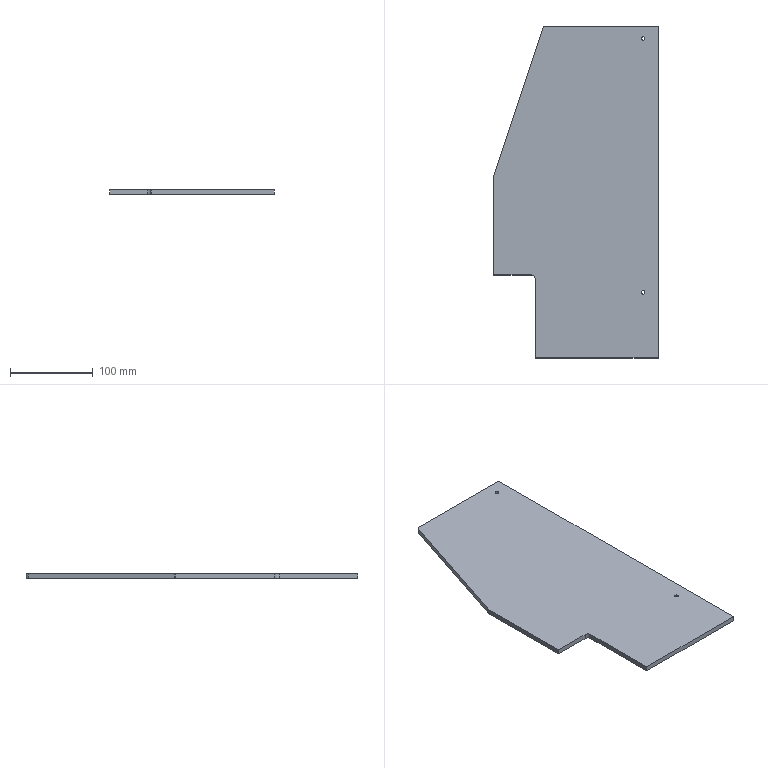Component | SolidWorks | THK-B1005LeftFrontBaffle-1 | 1 solid | 16 faces | box 198 x 400 x 6 mm | volume 412657 mm3 | plane 9 | cylinder 7 | commonest cylinder face diameters 4.2 x4 8 x2 10 x1 | material Q235A
build123d program:
from build123d import *

# Parameters (mm, degrees)
BOSS_EXTRUDE1_DEPTH = 3
M5_TAPPED_HOLE1_D   = 4.2
FILLET1_R           = 4


with BuildPart() as part:
    # Sketch1 → Boss-Extrude1 (new, symmetric)
    with BuildSketch(Plane.XY):
        with BuildLine():
            Line((-39, 200), (99, 200))
            Line((99, 200), (99, -200))
            Line((99, -200), (-49, -200))
            Line((-49, -200), (-49, -105))
            ThreePointArc((-49, -105), (-50.464, -101.464), (-54, -100))
            Line((-54, -100), (-99, -100))
            Line((-99, -100), (-99, 20))
            Line((-99, 20), (-39, 200))
        make_face()
    extrude(amount=BOSS_EXTRUDE1_DEPTH, both=True)

    # M5 Tapped Hole1 (through all)
    with Locations(Plane.XY.offset(3)):
        with Locations((81, 185), (81, -121)):
            Hole(M5_TAPPED_HOLE1_D / 2)

    # Fillet1
    fillet1_edges = [part.edges().sort_by_distance(p)[0] for p in [
        (-99, 20, 0),
        (-39, 200, 0),
    ]]
    fillet(fillet1_edges, radius=FILLET1_R)


solid = part.part

# Placed as in the assembly
solid = solid.moved(Location((-221, 0, -258), (0, 0, 0)))
STEP:
#1=COLOUR_RGB('',0.7922,0.8196,0.9333);
#2=FILL_AREA_STYLE_COLOUR('',#1);
#3=FILL_AREA_STYLE('',(#2));
#4=SURFACE_STYLE_FILL_AREA(#3);
#5=SURFACE_SIDE_STYLE('',(#4));
#6=SURFACE_STYLE_USAGE(.BOTH.,#5);
#7=PRESENTATION_STYLE_ASSIGNMENT((#6));
#8=CARTESIAN_POINT('',(-5.594,7.283,-10.276));
#9=VERTEX_POINT('',#8);
#10=CARTESIAN_POINT('',(-5.429,7.283,-10.276));
#11=VERTEX_POINT('',#10);
#12=CARTESIAN_POINT('',(-5.512,7.283,-10.276));
#13=DIRECTION('',(0.,0.,1.));
#14=DIRECTION('',(1.,0.,0.));
#15=AXIS2_PLACEMENT_3D('',#12,#13,#14);
#16=CIRCLE('',#15,0.08268);
#17=EDGE_CURVE('',#9,#11,#16,.T.);
#18=ORIENTED_EDGE('',*,*,#17,.F.);
#19=CARTESIAN_POINT('',(-5.594,7.283,-10.039));
#20=VERTEX_POINT('',#19);
#21=CARTESIAN_POINT('',(-5.594,7.283,-10.039));
#22=DIRECTION('',(0.,0.,1.));
#23=VECTOR('',#22,39.37);
#24=LINE('',#21,#23);
#25=EDGE_CURVE('',#9,#20,#24,.T.);
#26=ORIENTED_EDGE('',*,*,#25,.T.);
#27=CARTESIAN_POINT('',(-5.429,7.283,-10.039));
#28=VERTEX_POINT('',#27);
#29=CARTESIAN_POINT('',(-5.512,7.283,-10.039));
#30=DIRECTION('',(0.,0.,1.));
#31=DIRECTION('',(1.,0.,0.));
#32=AXIS2_PLACEMENT_3D('',#29,#30,#31);
#33=CIRCLE('',#32,0.08268);
#34=EDGE_CURVE('',#20,#28,#33,.T.);
#35=ORIENTED_EDGE('',*,*,#34,.T.);
#36=CARTESIAN_POINT('',(-5.429,7.283,-10.039));
#37=DIRECTION('',(0.,0.,1.));
#38=VECTOR('',#37,39.37);
#39=LINE('',#36,#38);
#40=EDGE_CURVE('',#11,#28,#39,.T.);
#41=ORIENTED_EDGE('',*,*,#40,.F.);
#42=EDGE_LOOP('',(#18,#26,#35,#41));
#43=FACE_OUTER_BOUND('',#42,.T.);
#44=CARTESIAN_POINT('',(-5.512,7.283,-10.039));
#45=DIRECTION('',(0.,0.,1.));
#46=DIRECTION('',(1.,0.,0.));
#47=AXIS2_PLACEMENT_3D('',#44,#45,#46);
#48=CYLINDRICAL_SURFACE('',#47,0.08268);
#49=ADVANCED_FACE('',(#43),#48,.F.);
#50=CARTESIAN_POINT('',(-5.594,-4.764,-10.276));
#51=VERTEX_POINT('',#50);
#52=CARTESIAN_POINT('',(-5.429,-4.764,-10.276));
#53=VERTEX_POINT('',#52);
#54=CARTESIAN_POINT('',(-5.512,-4.764,-10.276));
#55=DIRECTION('',(0.,0.,1.));
#56=DIRECTION('',(1.,0.,0.));
#57=AXIS2_PLACEMENT_3D('',#54,#55,#56);
#58=CIRCLE('',#57,0.08268);
#59=EDGE_CURVE('',#51,#53,#58,.T.);
#60=ORIENTED_EDGE('',*,*,#59,.F.);
#61=CARTESIAN_POINT('',(-5.594,-4.764,-10.039));
#62=VERTEX_POINT('',#61);
#63=CARTESIAN_POINT('',(-5.594,-4.764,-10.039));
#64=DIRECTION('',(0.,0.,1.));
#65=VECTOR('',#64,39.37);
#66=LINE('',#63,#65);
#67=EDGE_CURVE('',#51,#62,#66,.T.);
#68=ORIENTED_EDGE('',*,*,#67,.T.);
#69=CARTESIAN_POINT('',(-5.429,-4.764,-10.039));
#70=VERTEX_POINT('',#69);
#71=CARTESIAN_POINT('',(-5.512,-4.764,-10.039));
#72=DIRECTION('',(0.,0.,1.));
#73=DIRECTION('',(1.,0.,0.));
#74=AXIS2_PLACEMENT_3D('',#71,#72,#73);
#75=CIRCLE('',#74,0.08268);
#76=EDGE_CURVE('',#62,#70,#75,.T.);
#77=ORIENTED_EDGE('',*,*,#76,.T.);
#78=CARTESIAN_POINT('',(-5.429,-4.764,-10.039));
#79=DIRECTION('',(0.,0.,1.));
#80=VECTOR('',#79,39.37);
#81=LINE('',#78,#80);
#82=EDGE_CURVE('',#53,#70,#81,.T.);
#83=ORIENTED_EDGE('',*,*,#82,.F.);
#84=EDGE_LOOP('',(#60,#68,#77,#83));
#85=FACE_OUTER_BOUND('',#84,.T.);
#86=CARTESIAN_POINT('',(-5.512,-4.764,-10.039));
#87=DIRECTION('',(0.,0.,1.));
#88=DIRECTION('',(1.,0.,0.));
#89=AXIS2_PLACEMENT_3D('',#86,#87,#88);
#90=CYLINDRICAL_SURFACE('',#89,0.08268);
#91=ADVANCED_FACE('',(#85),#90,.F.);
#92=CARTESIAN_POINT('',(-12.598,0.7618,-10.039));
#93=VERTEX_POINT('',#92);
#94=CARTESIAN_POINT('',(-12.598,-3.937,-10.039));
#95=VERTEX_POINT('',#94);
#96=CARTESIAN_POINT('',(-12.598,0.7874,-10.039));
#97=DIRECTION('',(0.,-1.,0.));
#98=VECTOR('',#97,39.37);
#99=LINE('',#96,#98);
#100=EDGE_CURVE('',#93,#95,#99,.T.);
#101=ORIENTED_EDGE('',*,*,#100,.F.);
#102=CARTESIAN_POINT('',(-12.598,0.7618,-10.276));
#103=VERTEX_POINT('',#102);
#104=CARTESIAN_POINT('',(-12.598,0.7618,-10.039));
#105=DIRECTION('',(0.,0.,-1.));
#106=VECTOR('',#105,39.37);
#107=LINE('',#104,#106);
#108=EDGE_CURVE('',#93,#103,#107,.T.);
#109=ORIENTED_EDGE('',*,*,#108,.T.);
#110=CARTESIAN_POINT('',(-12.598,-3.937,-10.276));
#111=VERTEX_POINT('',#110);
#112=CARTESIAN_POINT('',(-12.598,0.7874,-10.276));
#113=DIRECTION('',(0.,-1.,0.));
#114=VECTOR('',#113,39.37);
#115=LINE('',#112,#114);
#116=EDGE_CURVE('',#103,#111,#115,.T.);
#117=ORIENTED_EDGE('',*,*,#116,.T.);
#118=CARTESIAN_POINT('',(-12.598,-3.937,-10.039));
#119=DIRECTION('',(0.,0.,-1.));
#120=VECTOR('',#119,39.37);
#121=LINE('',#118,#120);
#122=EDGE_CURVE('',#95,#111,#121,.T.);
#123=ORIENTED_EDGE('',*,*,#122,.F.);
#124=EDGE_LOOP('',(#101,#109,#117,#123));
#125=FACE_OUTER_BOUND('',#124,.T.);
#126=CARTESIAN_POINT('',(-12.598,0.7874,-10.039));
#127=DIRECTION('',(1.,0.,0.));
#128=DIRECTION('',(0.,0.,-1.));
#129=AXIS2_PLACEMENT_3D('',#126,#127,#128);
#130=PLANE('',#129);
#131=ADVANCED_FACE('',(#125),#130,.F.);
#132=CARTESIAN_POINT('',(-10.827,-3.937,-10.276));
#133=VERTEX_POINT('',#132);
#134=CARTESIAN_POINT('',(-10.827,-3.937,-10.276));
#135=DIRECTION('',(1.,0.,0.));
#136=VECTOR('',#135,39.37);
#137=LINE('',#134,#136);
#138=EDGE_CURVE('',#111,#133,#137,.T.);
#139=ORIENTED_EDGE('',*,*,#138,.T.);
#140=CARTESIAN_POINT('',(-10.827,-3.937,-10.039));
#141=VERTEX_POINT('',#140);
#142=CARTESIAN_POINT('',(-10.827,-3.937,-10.039));
#143=DIRECTION('',(0.,0.,-1.));
#144=VECTOR('',#143,39.37);
#145=LINE('',#142,#144);
#146=EDGE_CURVE('',#141,#133,#145,.T.);
#147=ORIENTED_EDGE('',*,*,#146,.F.);
#148=CARTESIAN_POINT('',(-10.827,-3.937,-10.039));
#149=DIRECTION('',(1.,0.,0.));
#150=VECTOR('',#149,39.37);
#151=LINE('',#148,#150);
#152=EDGE_CURVE('',#95,#141,#151,.T.);
#153=ORIENTED_EDGE('',*,*,#152,.F.);
#154=ORIENTED_EDGE('',*,*,#122,.T.);
#155=EDGE_LOOP('',(#139,#147,#153,#154));
#156=FACE_OUTER_BOUND('',#155,.T.);
#157=CARTESIAN_POINT('',(-10.827,-3.937,-10.039));
#158=DIRECTION('',(-0.,1.,0.));
#159=DIRECTION('',(-1.,-0.,0.));
#160=AXIS2_PLACEMENT_3D('',#157,#158,#159);
#161=PLANE('',#160);
#162=ADVANCED_FACE('',(#156),#161,.F.);
#163=CARTESIAN_POINT('',(-10.63,-4.134,-10.276));
#164=VERTEX_POINT('',#163);
#165=CARTESIAN_POINT('',(-10.827,-4.134,-10.276));
#166=DIRECTION('',(0.,0.,-1.));
#167=DIRECTION('',(1.,0.,0.));
#168=AXIS2_PLACEMENT_3D('',#165,#166,#167);
#169=CIRCLE('',#168,0.1969);
#170=EDGE_CURVE('',#133,#164,#169,.T.);
#171=ORIENTED_EDGE('',*,*,#170,.T.);
#172=CARTESIAN_POINT('',(-10.63,-4.134,-10.039));
#173=VERTEX_POINT('',#172);
#174=CARTESIAN_POINT('',(-10.63,-4.134,-10.039));
#175=DIRECTION('',(0.,0.,-1.));
#176=VECTOR('',#175,39.37);
#177=LINE('',#174,#176);
#178=EDGE_CURVE('',#173,#164,#177,.T.);
#179=ORIENTED_EDGE('',*,*,#178,.F.);
#180=CARTESIAN_POINT('',(-10.827,-4.134,-10.039));
#181=DIRECTION('',(0.,0.,-1.));
#182=DIRECTION('',(1.,0.,0.));
#183=AXIS2_PLACEMENT_3D('',#180,#181,#182);
#184=CIRCLE('',#183,0.1969);
#185=EDGE_CURVE('',#141,#173,#184,.T.);
#186=ORIENTED_EDGE('',*,*,#185,.F.);
#187=ORIENTED_EDGE('',*,*,#146,.T.);
#188=EDGE_LOOP('',(#171,#179,#186,#187));
#189=FACE_OUTER_BOUND('',#188,.T.);
#190=CARTESIAN_POINT('',(-10.827,-4.134,-10.039));
#191=DIRECTION('',(0.,0.,-1.));
#192=DIRECTION('',(-1.,0.,0.));
#193=AXIS2_PLACEMENT_3D('',#190,#191,#192);
#194=CYLINDRICAL_SURFACE('',#193,0.1969);
#195=ADVANCED_FACE('',(#189),#194,.F.);
#196=CARTESIAN_POINT('',(-10.63,-7.874,-10.276));
#197=VERTEX_POINT('',#196);
#198=CARTESIAN_POINT('',(-10.63,-7.874,-10.276));
#199=DIRECTION('',(0.,-1.,0.));
#200=VECTOR('',#199,39.37);
#201=LINE('',#198,#200);
#202=EDGE_CURVE('',#164,#197,#201,.T.);
#203=ORIENTED_EDGE('',*,*,#202,.T.);
#204=CARTESIAN_POINT('',(-10.63,-7.874,-10.039));
#205=VERTEX_POINT('',#204);
#206=CARTESIAN_POINT('',(-10.63,-7.874,-10.039));
#207=DIRECTION('',(0.,0.,-1.));
#208=VECTOR('',#207,39.37);
#209=LINE('',#206,#208);
#210=EDGE_CURVE('',#205,#197,#209,.T.);
#211=ORIENTED_EDGE('',*,*,#210,.F.);
#212=CARTESIAN_POINT('',(-10.63,-7.874,-10.039));
#213=DIRECTION('',(0.,-1.,0.));
#214=VECTOR('',#213,39.37);
#215=LINE('',#212,#214);
#216=EDGE_CURVE('',#173,#205,#215,.T.);
#217=ORIENTED_EDGE('',*,*,#216,.F.);
#218=ORIENTED_EDGE('',*,*,#178,.T.);
#219=EDGE_LOOP('',(#203,#211,#217,#218));
#220=FACE_OUTER_BOUND('',#219,.T.);
#221=CARTESIAN_POINT('',(-10.63,-7.874,-10.039));
#222=DIRECTION('',(1.,0.,0.));
#223=DIRECTION('',(0.,0.,-1.));
#224=AXIS2_PLACEMENT_3D('',#221,#222,#223);
#225=PLANE('',#224);
#226=ADVANCED_FACE('',(#220),#225,.F.);
#227=CARTESIAN_POINT('',(-4.803,-7.874,-10.276));
#228=VERTEX_POINT('',#227);
#229=CARTESIAN_POINT('',(-10.63,-7.874,-10.276));
#230=DIRECTION('',(1.,0.,0.));
#231=VECTOR('',#230,39.37);
#232=LINE('',#229,#231);
#233=EDGE_CURVE('',#197,#228,#232,.T.);
#234=ORIENTED_EDGE('',*,*,#233,.T.);
#235=CARTESIAN_POINT('',(-4.803,-7.874,-10.039));
#236=VERTEX_POINT('',#235);
#237=CARTESIAN_POINT('',(-4.803,-7.874,-10.039));
#238=DIRECTION('',(0.,0.,-1.));
#239=VECTOR('',#238,39.37);
#240=LINE('',#237,#239);
#241=EDGE_CURVE('',#236,#228,#240,.T.);
#242=ORIENTED_EDGE('',*,*,#241,.F.);
#243=CARTESIAN_POINT('',(-10.63,-7.874,-10.039));
#244=DIRECTION('',(1.,0.,0.));
#245=VECTOR('',#244,39.37);
#246=LINE('',#243,#245);
#247=EDGE_CURVE('',#205,#236,#246,.T.);
#248=ORIENTED_EDGE('',*,*,#247,.F.);
#249=ORIENTED_EDGE('',*,*,#210,.T.);
#250=EDGE_LOOP('',(#234,#242,#248,#249));
#251=FACE_OUTER_BOUND('',#250,.T.);
#252=CARTESIAN_POINT('',(-10.63,-7.874,-10.039));
#253=DIRECTION('',(0.,1.,0.));
#254=DIRECTION('',(0.,0.,1.));
#255=AXIS2_PLACEMENT_3D('',#252,#253,#254);
#256=PLANE('',#255);
#257=ADVANCED_FACE('',(#251),#256,.F.);
#258=CARTESIAN_POINT('',(-4.803,7.874,-10.276));
#259=VERTEX_POINT('',#258);
#260=CARTESIAN_POINT('',(-4.803,7.874,-10.276));
#261=DIRECTION('',(0.,1.,0.));
#262=VECTOR('',#261,39.37);
#263=LINE('',#260,#262);
#264=EDGE_CURVE('',#228,#259,#263,.T.);
#265=ORIENTED_EDGE('',*,*,#264,.T.);
#266=CARTESIAN_POINT('',(-4.803,7.874,-10.039));
#267=VERTEX_POINT('',#266);
#268=CARTESIAN_POINT('',(-4.803,7.874,-10.039));
#269=DIRECTION('',(0.,0.,-1.));
#270=VECTOR('',#269,39.37);
#271=LINE('',#268,#270);
#272=EDGE_CURVE('',#267,#259,#271,.T.);
#273=ORIENTED_EDGE('',*,*,#272,.F.);
#274=CARTESIAN_POINT('',(-4.803,7.874,-10.039));
#275=DIRECTION('',(0.,1.,0.));
#276=VECTOR('',#275,39.37);
#277=LINE('',#274,#276);
#278=EDGE_CURVE('',#236,#267,#277,.T.);
#279=ORIENTED_EDGE('',*,*,#278,.F.);
#280=ORIENTED_EDGE('',*,*,#241,.T.);
#281=EDGE_LOOP('',(#265,#273,#279,#280));
#282=FACE_OUTER_BOUND('',#281,.T.);
#283=CARTESIAN_POINT('',(-4.803,7.874,-10.039));
#284=DIRECTION('',(-1.,0.,0.));
#285=DIRECTION('',(0.,0.,1.));
#286=AXIS2_PLACEMENT_3D('',#283,#284,#285);
#287=PLANE('',#286);
#288=ADVANCED_FACE('',(#282),#287,.F.);
#289=CARTESIAN_POINT('',(-10.123,7.874,-10.276));
#290=VERTEX_POINT('',#289);
#291=CARTESIAN_POINT('',(-10.236,7.874,-10.276));
#292=DIRECTION('',(-1.,0.,0.));
#293=VECTOR('',#292,39.37);
#294=LINE('',#291,#293);
#295=EDGE_CURVE('',#259,#290,#294,.T.);
#296=ORIENTED_EDGE('',*,*,#295,.T.);
#297=CARTESIAN_POINT('',(-10.123,7.874,-10.039));
#298=VERTEX_POINT('',#297);
#299=CARTESIAN_POINT('',(-10.123,7.874,-10.039));
#300=DIRECTION('',(0.,0.,1.));
#301=VECTOR('',#300,39.37);
#302=LINE('',#299,#301);
#303=EDGE_CURVE('',#290,#298,#302,.T.);
#304=ORIENTED_EDGE('',*,*,#303,.T.);
#305=CARTESIAN_POINT('',(-10.236,7.874,-10.039));
#306=DIRECTION('',(-1.,0.,0.));
#307=VECTOR('',#306,39.37);
#308=LINE('',#305,#307);
#309=EDGE_CURVE('',#267,#298,#308,.T.);
#310=ORIENTED_EDGE('',*,*,#309,.F.);
#311=ORIENTED_EDGE('',*,*,#272,.T.);
#312=EDGE_LOOP('',(#296,#304,#310,#311));
#313=FACE_OUTER_BOUND('',#312,.T.);
#314=CARTESIAN_POINT('',(-10.236,7.874,-10.039));
#315=DIRECTION('',(0.,-1.,0.));
#316=DIRECTION('',(0.,0.,-1.));
#317=AXIS2_PLACEMENT_3D('',#314,#315,#316);
#318=PLANE('',#317);
#319=ADVANCED_FACE('',(#313),#318,.F.);
#320=CARTESIAN_POINT('',(-10.272,7.766,-10.276));
#321=VERTEX_POINT('',#320);
#322=CARTESIAN_POINT('',(-12.59,0.8116,-10.276));
#323=VERTEX_POINT('',#322);
#324=CARTESIAN_POINT('',(-10.236,7.874,-10.276));
#325=DIRECTION('',(-0.3162,-0.9487,0.));
#326=VECTOR('',#325,39.37);
#327=LINE('',#324,#326);
#328=EDGE_CURVE('',#321,#323,#327,.T.);
#329=ORIENTED_EDGE('',*,*,#328,.T.);
#330=CARTESIAN_POINT('',(-12.59,0.8116,-10.039));
#331=VERTEX_POINT('',#330);
#332=CARTESIAN_POINT('',(-12.59,0.8116,-10.039));
#333=DIRECTION('',(0.,0.,1.));
#334=VECTOR('',#333,39.37);
#335=LINE('',#332,#334);
#336=EDGE_CURVE('',#323,#331,#335,.T.);
#337=ORIENTED_EDGE('',*,*,#336,.T.);
#338=CARTESIAN_POINT('',(-10.272,7.766,-10.039));
#339=VERTEX_POINT('',#338);
#340=CARTESIAN_POINT('',(-10.236,7.874,-10.039));
#341=DIRECTION('',(-0.3162,-0.9487,0.));
#342=VECTOR('',#341,39.37);
#343=LINE('',#340,#342);
#344=EDGE_CURVE('',#339,#331,#343,.T.);
#345=ORIENTED_EDGE('',*,*,#344,.F.);
#346=CARTESIAN_POINT('',(-10.272,7.766,-10.039));
#347=DIRECTION('',(0.,0.,-1.));
#348=VECTOR('',#347,39.37);
#349=LINE('',#346,#348);
#350=EDGE_CURVE('',#339,#321,#349,.T.);
#351=ORIENTED_EDGE('',*,*,#350,.T.);
#352=EDGE_LOOP('',(#329,#337,#345,#351));
#353=FACE_OUTER_BOUND('',#352,.T.);
#354=CARTESIAN_POINT('',(-10.236,7.874,-10.039));
#355=DIRECTION('',(0.9487,-0.3162,0.));
#356=DIRECTION('',(0.3162,0.9487,0.));
#357=AXIS2_PLACEMENT_3D('',#354,#355,#356);
#358=PLANE('',#357);
#359=ADVANCED_FACE('',(#353),#358,.F.);
#360=CARTESIAN_POINT('',(-5.512,7.283,-10.039));
#361=DIRECTION('',(0.,0.,1.));
#362=DIRECTION('',(1.,0.,0.));
#363=AXIS2_PLACEMENT_3D('',#360,#361,#362);
#364=CIRCLE('',#363,0.08268);
#365=EDGE_CURVE('',#28,#20,#364,.T.);
#366=ORIENTED_EDGE('',*,*,#365,.F.);
#367=ORIENTED_EDGE('',*,*,#34,.F.);
#368=EDGE_LOOP('',(#366,#367));
#369=FACE_BOUND('',#368,.T.);
#370=CARTESIAN_POINT('',(-5.512,-4.764,-10.039));
#371=DIRECTION('',(0.,0.,1.));
#372=DIRECTION('',(1.,0.,0.));
#373=AXIS2_PLACEMENT_3D('',#370,#371,#372);
#374=CIRCLE('',#373,0.08268);
#375=EDGE_CURVE('',#70,#62,#374,.T.);
#376=ORIENTED_EDGE('',*,*,#375,.F.);
#377=ORIENTED_EDGE('',*,*,#76,.F.);
#378=EDGE_LOOP('',(#376,#377));
#379=FACE_BOUND('',#378,.T.);
#380=ORIENTED_EDGE('',*,*,#344,.T.);
#381=CARTESIAN_POINT('',(-12.441,0.7618,-10.039));
#382=DIRECTION('',(0.,0.,1.));
#383=DIRECTION('',(1.,0.,0.));
#384=AXIS2_PLACEMENT_3D('',#381,#382,#383);
#385=CIRCLE('',#384,0.1575);
#386=EDGE_CURVE('',#331,#93,#385,.T.);
#387=ORIENTED_EDGE('',*,*,#386,.T.);
#388=ORIENTED_EDGE('',*,*,#100,.T.);
#389=ORIENTED_EDGE('',*,*,#152,.T.);
#390=ORIENTED_EDGE('',*,*,#185,.T.);
#391=ORIENTED_EDGE('',*,*,#216,.T.);
#392=ORIENTED_EDGE('',*,*,#247,.T.);
#393=ORIENTED_EDGE('',*,*,#278,.T.);
#394=ORIENTED_EDGE('',*,*,#309,.T.);
#395=CARTESIAN_POINT('',(-10.123,7.717,-10.039));
#396=DIRECTION('',(0.,0.,1.));
#397=DIRECTION('',(1.,0.,0.));
#398=AXIS2_PLACEMENT_3D('',#395,#396,#397);
#399=CIRCLE('',#398,0.1575);
#400=EDGE_CURVE('',#298,#339,#399,.T.);
#401=ORIENTED_EDGE('',*,*,#400,.T.);
#402=EDGE_LOOP('',(#380,#387,#388,#389,#390,#391,#392,#393,#394,#401));
#403=FACE_OUTER_BOUND('',#402,.T.);
#404=CARTESIAN_POINT('',(-10.827,-4.134,-10.039));
#405=DIRECTION('',(0.,0.,1.));
#406=DIRECTION('',(1.,0.,0.));
#407=AXIS2_PLACEMENT_3D('',#404,#405,#406);
#408=PLANE('',#407);
#409=ADVANCED_FACE('',(#369,#379,#403),#408,.T.);
#410=CARTESIAN_POINT('',(-5.512,7.283,-10.276));
#411=DIRECTION('',(0.,0.,1.));
#412=DIRECTION('',(1.,0.,0.));
#413=AXIS2_PLACEMENT_3D('',#410,#411,#412);
#414=CIRCLE('',#413,0.08268);
#415=EDGE_CURVE('',#11,#9,#414,.T.);
#416=ORIENTED_EDGE('',*,*,#415,.T.);
#417=ORIENTED_EDGE('',*,*,#17,.T.);
#418=EDGE_LOOP('',(#416,#417));
#419=FACE_BOUND('',#418,.T.);
#420=CARTESIAN_POINT('',(-5.512,-4.764,-10.276));
#421=DIRECTION('',(0.,0.,1.));
#422=DIRECTION('',(1.,0.,0.));
#423=AXIS2_PLACEMENT_3D('',#420,#421,#422);
#424=CIRCLE('',#423,0.08268);
#425=EDGE_CURVE('',#53,#51,#424,.T.);
#426=ORIENTED_EDGE('',*,*,#425,.T.);
#427=ORIENTED_EDGE('',*,*,#59,.T.);
#428=EDGE_LOOP('',(#426,#427));
#429=FACE_BOUND('',#428,.T.);
#430=ORIENTED_EDGE('',*,*,#116,.F.);
#431=CARTESIAN_POINT('',(-12.441,0.7618,-10.276));
#432=DIRECTION('',(0.,0.,-1.));
#433=DIRECTION('',(1.,0.,0.));
#434=AXIS2_PLACEMENT_3D('',#431,#432,#433);
#435=CIRCLE('',#434,0.1575);
#436=EDGE_CURVE('',#103,#323,#435,.T.);
#437=ORIENTED_EDGE('',*,*,#436,.T.);
#438=ORIENTED_EDGE('',*,*,#328,.F.);
#439=CARTESIAN_POINT('',(-10.123,7.717,-10.276));
#440=DIRECTION('',(0.,0.,-1.));
#441=DIRECTION('',(1.,0.,0.));
#442=AXIS2_PLACEMENT_3D('',#439,#440,#441);
#443=CIRCLE('',#442,0.1575);
#444=EDGE_CURVE('',#321,#290,#443,.T.);
#445=ORIENTED_EDGE('',*,*,#444,.T.);
#446=ORIENTED_EDGE('',*,*,#295,.F.);
#447=ORIENTED_EDGE('',*,*,#264,.F.);
#448=ORIENTED_EDGE('',*,*,#233,.F.);
#449=ORIENTED_EDGE('',*,*,#202,.F.);
#450=ORIENTED_EDGE('',*,*,#170,.F.);
#451=ORIENTED_EDGE('',*,*,#138,.F.);
#452=EDGE_LOOP('',(#430,#437,#438,#445,#446,#447,#448,#449,#450,#451));
#453=FACE_OUTER_BOUND('',#452,.T.);
#454=CARTESIAN_POINT('',(-10.827,-4.134,-10.276));
#455=DIRECTION('',(0.,0.,1.));
#456=DIRECTION('',(1.,0.,0.));
#457=AXIS2_PLACEMENT_3D('',#454,#455,#456);
#458=PLANE('',#457);
#459=ADVANCED_FACE('',(#419,#429,#453),#458,.F.);
#460=ORIENTED_EDGE('',*,*,#67,.F.);
#461=ORIENTED_EDGE('',*,*,#425,.F.);
#462=ORIENTED_EDGE('',*,*,#82,.T.);
#463=ORIENTED_EDGE('',*,*,#375,.T.);
#464=EDGE_LOOP('',(#460,#461,#462,#463));
#465=FACE_OUTER_BOUND('',#464,.T.);
#466=CARTESIAN_POINT('',(-5.512,-4.764,-10.039));
#467=DIRECTION('',(0.,0.,1.));
#468=DIRECTION('',(1.,0.,0.));
#469=AXIS2_PLACEMENT_3D('',#466,#467,#468);
#470=CYLINDRICAL_SURFACE('',#469,0.08268);
#471=ADVANCED_FACE('',(#465),#470,.F.);
#472=ORIENTED_EDGE('',*,*,#25,.F.);
#473=ORIENTED_EDGE('',*,*,#415,.F.);
#474=ORIENTED_EDGE('',*,*,#40,.T.);
#475=ORIENTED_EDGE('',*,*,#365,.T.);
#476=EDGE_LOOP('',(#472,#473,#474,#475));
#477=FACE_OUTER_BOUND('',#476,.T.);
#478=CARTESIAN_POINT('',(-5.512,7.283,-10.039));
#479=DIRECTION('',(0.,0.,1.));
#480=DIRECTION('',(1.,0.,0.));
#481=AXIS2_PLACEMENT_3D('',#478,#479,#480);
#482=CYLINDRICAL_SURFACE('',#481,0.08268);
#483=ADVANCED_FACE('',(#477),#482,.F.);
#484=ORIENTED_EDGE('',*,*,#386,.F.);
#485=ORIENTED_EDGE('',*,*,#336,.F.);
#486=ORIENTED_EDGE('',*,*,#436,.F.);
#487=ORIENTED_EDGE('',*,*,#108,.F.);
#488=EDGE_LOOP('',(#484,#485,#486,#487));
#489=FACE_OUTER_BOUND('',#488,.T.);
#490=CARTESIAN_POINT('',(-12.441,0.7618,-10.039));
#491=DIRECTION('',(0.,0.,-1.));
#492=DIRECTION('',(-1.,0.,0.));
#493=AXIS2_PLACEMENT_3D('',#490,#491,#492);
#494=CYLINDRICAL_SURFACE('',#493,0.1575);
#495=ADVANCED_FACE('',(#489),#494,.T.);
#496=ORIENTED_EDGE('',*,*,#400,.F.);
#497=ORIENTED_EDGE('',*,*,#303,.F.);
#498=ORIENTED_EDGE('',*,*,#444,.F.);
#499=ORIENTED_EDGE('',*,*,#350,.F.);
#500=EDGE_LOOP('',(#496,#497,#498,#499));
#501=FACE_OUTER_BOUND('',#500,.T.);
#502=CARTESIAN_POINT('',(-10.123,7.717,-10.039));
#503=DIRECTION('',(0.,0.,-1.));
#504=DIRECTION('',(-1.,0.,0.));
#505=AXIS2_PLACEMENT_3D('',#502,#503,#504);
#506=CYLINDRICAL_SURFACE('',#505,0.1575);
#507=ADVANCED_FACE('',(#501),#506,.T.);
#508=CLOSED_SHELL('',(#49,#91,#131,#162,#195,#226,#257,#288,#319,#359,#409,#459,#471,#483,#495,#507));
#509=MANIFOLD_SOLID_BREP('',#508);
#510=STYLED_ITEM('',(#7),#509);
#511=(LENGTH_UNIT()NAMED_UNIT(*)SI_UNIT($,.METRE.));
#512=LENGTH_MEASURE_WITH_UNIT(LENGTH_MEASURE(0.0254),#511);
#513=DIMENSIONAL_EXPONENTS(1.,0.,0.,0.,0.,0.,0.);
#514=(CONVERSION_BASED_UNIT('',#512)LENGTH_UNIT()NAMED_UNIT(#513));
#515=UNCERTAINTY_MEASURE_WITH_UNIT(LENGTH_MEASURE(0.00001),#514,'','');
#516=(NAMED_UNIT(*)PLANE_ANGLE_UNIT()SI_UNIT($,.RADIAN.));
#517=(NAMED_UNIT(*)SI_UNIT($,.STERADIAN.)SOLID_ANGLE_UNIT());
#518=(GEOMETRIC_REPRESENTATION_CONTEXT(3)GLOBAL_UNCERTAINTY_ASSIGNED_CONTEXT((#515))GLOBAL_UNIT_ASSIGNED_CONTEXT((#514,#516,#517))REPRESENTATION_CONTEXT('',''));
#519=MECHANICAL_DESIGN_GEOMETRIC_PRESENTATION_REPRESENTATION('',(#510),#518);
#520=CARTESIAN_POINT('',(0.,0.,0.));
#521=DIRECTION('',(0.,0.,1.));
#522=DIRECTION('',(1.,0.,0.));
#523=AXIS2_PLACEMENT_3D('',#520,#521,#522);
#524=(LENGTH_UNIT()NAMED_UNIT(*)SI_UNIT($,.METRE.));
#525=LENGTH_MEASURE_WITH_UNIT(LENGTH_MEASURE(0.0254),#524);
#526=DIMENSIONAL_EXPONENTS(1.,0.,0.,0.,0.,0.,0.);
#527=(CONVERSION_BASED_UNIT('',#525)LENGTH_UNIT()NAMED_UNIT(#526));
#528=UNCERTAINTY_MEASURE_WITH_UNIT(LENGTH_MEASURE(0.00001),#527,'','');
#529=(NAMED_UNIT(*)PLANE_ANGLE_UNIT()SI_UNIT($,.RADIAN.));
#530=(NAMED_UNIT(*)SI_UNIT($,.STERADIAN.)SOLID_ANGLE_UNIT());
#531=(GEOMETRIC_REPRESENTATION_CONTEXT(3)GLOBAL_UNCERTAINTY_ASSIGNED_CONTEXT((#528))GLOBAL_UNIT_ASSIGNED_CONTEXT((#527,#529,#530))REPRESENTATION_CONTEXT('',''));
#532=ADVANCED_BREP_SHAPE_REPRESENTATION('',(#509,#523),#531);
#533=PRESENTATION_LAYER_ASSIGNMENT('','',(#510));